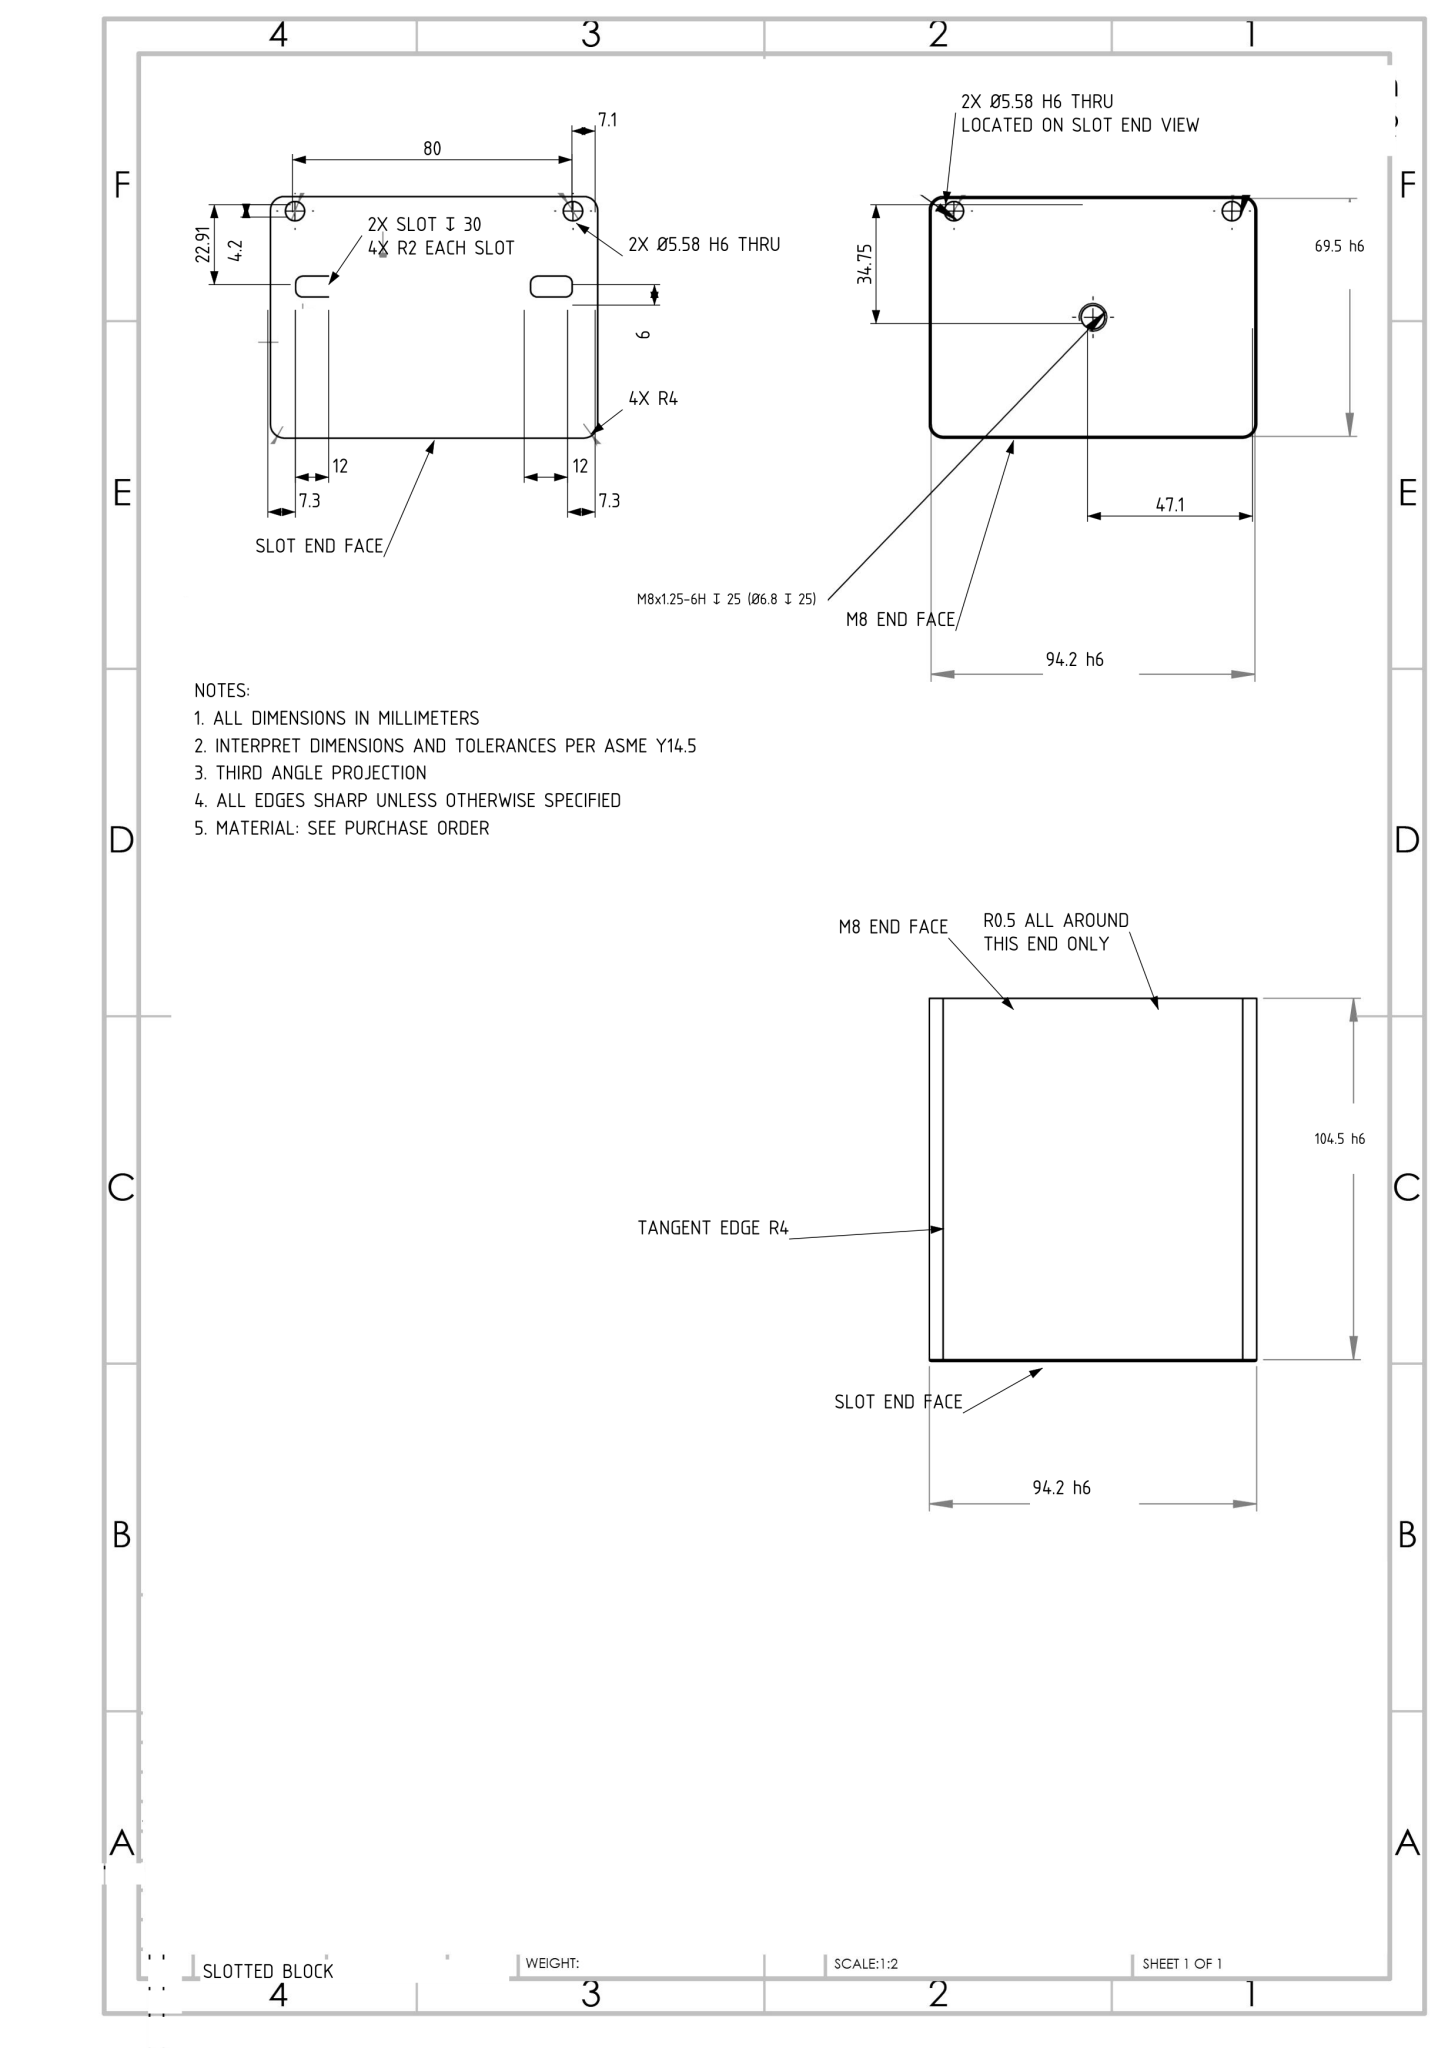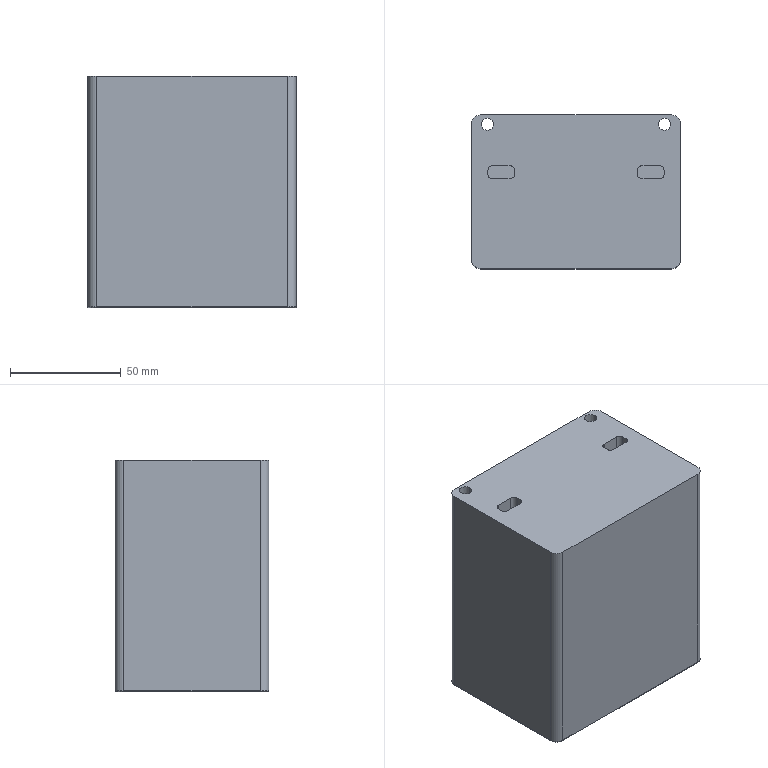Part | NX | mm | 1 solid | 43 faces | box 94.2 x 69.5 x 104.5 mm | volume 672566 mm3 | cylinder 22 | plane 17 | torus 4 | commonest cylinder face diameters 4 x8 5.58 x4 8 x4 1 x4 6.8 x2